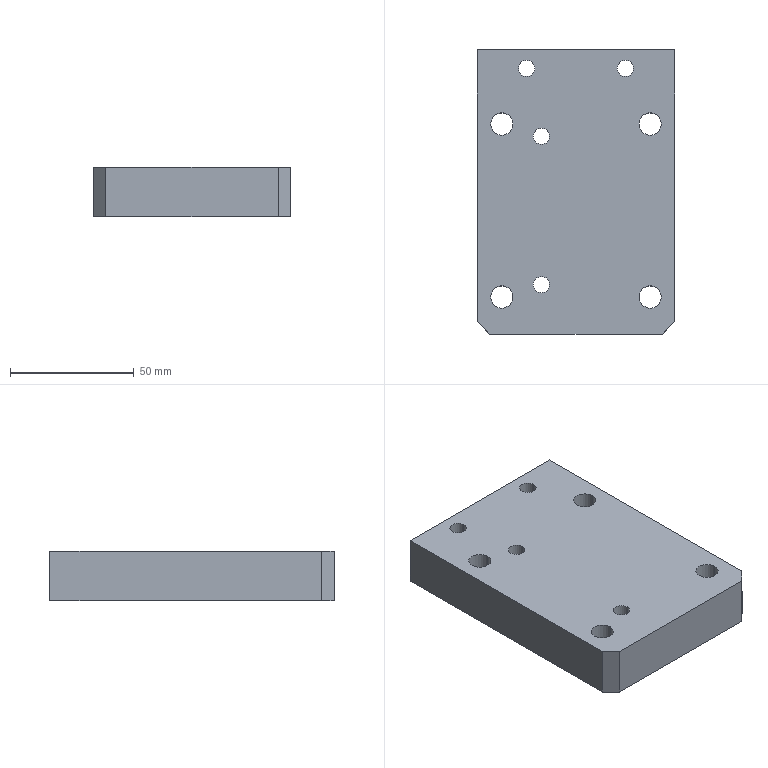Component | SolidWorks | 8TC-A15004-80-02A-2 | 1 solid | 36 faces | box 80 x 115 x 20 mm | volume 174117 mm3 | cylinder 24 | plane 12 | commonest cylinder face diameters 9 x8 11 x8 6.6 x8 | material A3
STEP:
#1=COLOUR_RGB('',0.7922,0.8196,0.9333);
#2=FILL_AREA_STYLE_COLOUR('',#1);
#3=FILL_AREA_STYLE('',(#2));
#4=SURFACE_STYLE_FILL_AREA(#3);
#5=SURFACE_SIDE_STYLE('',(#4));
#6=SURFACE_STYLE_USAGE(.BOTH.,#5);
#7=PRESENTATION_STYLE_ASSIGNMENT((#6));
#8=CARTESIAN_POINT('',(0.2165,-3.642,0.7874));
#9=VERTEX_POINT('',#8);
#10=CARTESIAN_POINT('',(0.5709,-3.642,0.7874));
#11=VERTEX_POINT('',#10);
#12=CARTESIAN_POINT('',(0.3937,-3.642,0.7874));
#13=DIRECTION('',(0.,0.,1.));
#14=DIRECTION('',(1.,0.,0.));
#15=AXIS2_PLACEMENT_3D('',#12,#13,#14);
#16=CIRCLE('',#15,0.1772);
#17=EDGE_CURVE('',#9,#11,#16,.T.);
#18=ORIENTED_EDGE('',*,*,#17,.F.);
#19=CARTESIAN_POINT('',(0.2165,-3.642,1.575));
#20=VERTEX_POINT('',#19);
#21=CARTESIAN_POINT('',(0.2165,-3.642,1.575));
#22=DIRECTION('',(0.,0.,1.));
#23=VECTOR('',#22,39.37);
#24=LINE('',#21,#23);
#25=EDGE_CURVE('',#9,#20,#24,.T.);
#26=ORIENTED_EDGE('',*,*,#25,.T.);
#27=CARTESIAN_POINT('',(0.5709,-3.642,1.575));
#28=VERTEX_POINT('',#27);
#29=CARTESIAN_POINT('',(0.3937,-3.642,1.575));
#30=DIRECTION('',(0.,0.,1.));
#31=DIRECTION('',(1.,0.,0.));
#32=AXIS2_PLACEMENT_3D('',#29,#30,#31);
#33=CIRCLE('',#32,0.1772);
#34=EDGE_CURVE('',#20,#28,#33,.T.);
#35=ORIENTED_EDGE('',*,*,#34,.T.);
#36=CARTESIAN_POINT('',(0.5709,-3.642,1.575));
#37=DIRECTION('',(0.,0.,1.));
#38=VECTOR('',#37,39.37);
#39=LINE('',#36,#38);
#40=EDGE_CURVE('',#11,#28,#39,.T.);
#41=ORIENTED_EDGE('',*,*,#40,.F.);
#42=EDGE_LOOP('',(#18,#26,#35,#41));
#43=FACE_OUTER_BOUND('',#42,.T.);
#44=CARTESIAN_POINT('',(0.3937,-3.642,1.575));
#45=DIRECTION('',(0.,0.,1.));
#46=DIRECTION('',(1.,0.,0.));
#47=AXIS2_PLACEMENT_3D('',#44,#45,#46);
#48=CYLINDRICAL_SURFACE('',#47,0.1772);
#49=ADVANCED_FACE('',(#43),#48,.F.);
#50=CARTESIAN_POINT('',(0.2165,-0.8858,0.7874));
#51=VERTEX_POINT('',#50);
#52=CARTESIAN_POINT('',(0.5709,-0.8858,0.7874));
#53=VERTEX_POINT('',#52);
#54=CARTESIAN_POINT('',(0.3937,-0.8858,0.7874));
#55=DIRECTION('',(0.,0.,1.));
#56=DIRECTION('',(1.,0.,0.));
#57=AXIS2_PLACEMENT_3D('',#54,#55,#56);
#58=CIRCLE('',#57,0.1772);
#59=EDGE_CURVE('',#51,#53,#58,.T.);
#60=ORIENTED_EDGE('',*,*,#59,.F.);
#61=CARTESIAN_POINT('',(0.2165,-0.8858,1.575));
#62=VERTEX_POINT('',#61);
#63=CARTESIAN_POINT('',(0.2165,-0.8858,1.575));
#64=DIRECTION('',(0.,0.,1.));
#65=VECTOR('',#64,39.37);
#66=LINE('',#63,#65);
#67=EDGE_CURVE('',#51,#62,#66,.T.);
#68=ORIENTED_EDGE('',*,*,#67,.T.);
#69=CARTESIAN_POINT('',(0.5709,-0.8858,1.575));
#70=VERTEX_POINT('',#69);
#71=CARTESIAN_POINT('',(0.3937,-0.8858,1.575));
#72=DIRECTION('',(0.,0.,1.));
#73=DIRECTION('',(1.,0.,0.));
#74=AXIS2_PLACEMENT_3D('',#71,#72,#73);
#75=CIRCLE('',#74,0.1772);
#76=EDGE_CURVE('',#62,#70,#75,.T.);
#77=ORIENTED_EDGE('',*,*,#76,.T.);
#78=CARTESIAN_POINT('',(0.5709,-0.8858,1.575));
#79=DIRECTION('',(0.,0.,1.));
#80=VECTOR('',#79,39.37);
#81=LINE('',#78,#80);
#82=EDGE_CURVE('',#53,#70,#81,.T.);
#83=ORIENTED_EDGE('',*,*,#82,.F.);
#84=EDGE_LOOP('',(#60,#68,#77,#83));
#85=FACE_OUTER_BOUND('',#84,.T.);
#86=CARTESIAN_POINT('',(0.3937,-0.8858,1.575));
#87=DIRECTION('',(0.,0.,1.));
#88=DIRECTION('',(1.,0.,0.));
#89=AXIS2_PLACEMENT_3D('',#86,#87,#88);
#90=CYLINDRICAL_SURFACE('',#89,0.1772);
#91=ADVANCED_FACE('',(#85),#90,.F.);
#92=CARTESIAN_POINT('',(2.579,-0.8858,0.7874));
#93=VERTEX_POINT('',#92);
#94=CARTESIAN_POINT('',(2.933,-0.8858,0.7874));
#95=VERTEX_POINT('',#94);
#96=CARTESIAN_POINT('',(2.756,-0.8858,0.7874));
#97=DIRECTION('',(0.,0.,1.));
#98=DIRECTION('',(1.,0.,0.));
#99=AXIS2_PLACEMENT_3D('',#96,#97,#98);
#100=CIRCLE('',#99,0.1772);
#101=EDGE_CURVE('',#93,#95,#100,.T.);
#102=ORIENTED_EDGE('',*,*,#101,.F.);
#103=CARTESIAN_POINT('',(2.579,-0.8858,1.575));
#104=VERTEX_POINT('',#103);
#105=CARTESIAN_POINT('',(2.579,-0.8858,1.575));
#106=DIRECTION('',(0.,0.,1.));
#107=VECTOR('',#106,39.37);
#108=LINE('',#105,#107);
#109=EDGE_CURVE('',#93,#104,#108,.T.);
#110=ORIENTED_EDGE('',*,*,#109,.T.);
#111=CARTESIAN_POINT('',(2.933,-0.8858,1.575));
#112=VERTEX_POINT('',#111);
#113=CARTESIAN_POINT('',(2.756,-0.8858,1.575));
#114=DIRECTION('',(0.,0.,1.));
#115=DIRECTION('',(1.,0.,0.));
#116=AXIS2_PLACEMENT_3D('',#113,#114,#115);
#117=CIRCLE('',#116,0.1772);
#118=EDGE_CURVE('',#104,#112,#117,.T.);
#119=ORIENTED_EDGE('',*,*,#118,.T.);
#120=CARTESIAN_POINT('',(2.933,-0.8858,1.575));
#121=DIRECTION('',(0.,0.,1.));
#122=VECTOR('',#121,39.37);
#123=LINE('',#120,#122);
#124=EDGE_CURVE('',#95,#112,#123,.T.);
#125=ORIENTED_EDGE('',*,*,#124,.F.);
#126=EDGE_LOOP('',(#102,#110,#119,#125));
#127=FACE_OUTER_BOUND('',#126,.T.);
#128=CARTESIAN_POINT('',(2.756,-0.8858,1.575));
#129=DIRECTION('',(0.,0.,1.));
#130=DIRECTION('',(1.,0.,0.));
#131=AXIS2_PLACEMENT_3D('',#128,#129,#130);
#132=CYLINDRICAL_SURFACE('',#131,0.1772);
#133=ADVANCED_FACE('',(#127),#132,.F.);
#134=CARTESIAN_POINT('',(2.579,-3.642,0.7874));
#135=VERTEX_POINT('',#134);
#136=CARTESIAN_POINT('',(2.933,-3.642,0.7874));
#137=VERTEX_POINT('',#136);
#138=CARTESIAN_POINT('',(2.756,-3.642,0.7874));
#139=DIRECTION('',(0.,0.,1.));
#140=DIRECTION('',(1.,0.,0.));
#141=AXIS2_PLACEMENT_3D('',#138,#139,#140);
#142=CIRCLE('',#141,0.1772);
#143=EDGE_CURVE('',#135,#137,#142,.T.);
#144=ORIENTED_EDGE('',*,*,#143,.F.);
#145=CARTESIAN_POINT('',(2.579,-3.642,1.575));
#146=VERTEX_POINT('',#145);
#147=CARTESIAN_POINT('',(2.579,-3.642,1.575));
#148=DIRECTION('',(0.,0.,1.));
#149=VECTOR('',#148,39.37);
#150=LINE('',#147,#149);
#151=EDGE_CURVE('',#135,#146,#150,.T.);
#152=ORIENTED_EDGE('',*,*,#151,.T.);
#153=CARTESIAN_POINT('',(2.933,-3.642,1.575));
#154=VERTEX_POINT('',#153);
#155=CARTESIAN_POINT('',(2.756,-3.642,1.575));
#156=DIRECTION('',(0.,0.,1.));
#157=DIRECTION('',(1.,0.,0.));
#158=AXIS2_PLACEMENT_3D('',#155,#156,#157);
#159=CIRCLE('',#158,0.1772);
#160=EDGE_CURVE('',#146,#154,#159,.T.);
#161=ORIENTED_EDGE('',*,*,#160,.T.);
#162=CARTESIAN_POINT('',(2.933,-3.642,1.575));
#163=DIRECTION('',(0.,0.,1.));
#164=VECTOR('',#163,39.37);
#165=LINE('',#162,#164);
#166=EDGE_CURVE('',#137,#154,#165,.T.);
#167=ORIENTED_EDGE('',*,*,#166,.F.);
#168=EDGE_LOOP('',(#144,#152,#161,#167));
#169=FACE_OUTER_BOUND('',#168,.T.);
#170=CARTESIAN_POINT('',(2.756,-3.642,1.575));
#171=DIRECTION('',(0.,0.,1.));
#172=DIRECTION('',(1.,0.,0.));
#173=AXIS2_PLACEMENT_3D('',#170,#171,#172);
#174=CYLINDRICAL_SURFACE('',#173,0.1772);
#175=ADVANCED_FACE('',(#169),#174,.F.);
#176=CARTESIAN_POINT('',(2.579,0.,1.039));
#177=VERTEX_POINT('',#176);
#178=CARTESIAN_POINT('',(2.146,0.,1.039));
#179=VERTEX_POINT('',#178);
#180=CARTESIAN_POINT('',(2.362,0.,1.039));
#181=DIRECTION('',(0.,0.,-1.));
#182=DIRECTION('',(-1.,0.,0.));
#183=AXIS2_PLACEMENT_3D('',#180,#181,#182);
#184=CIRCLE('',#183,0.2165);
#185=EDGE_CURVE('',#177,#179,#184,.T.);
#186=ORIENTED_EDGE('',*,*,#185,.F.);
#187=CARTESIAN_POINT('',(2.579,0.,0.7874));
#188=VERTEX_POINT('',#187);
#189=CARTESIAN_POINT('',(2.579,0.,0.7874));
#190=DIRECTION('',(0.,0.,-1.));
#191=VECTOR('',#190,39.37);
#192=LINE('',#189,#191);
#193=EDGE_CURVE('',#177,#188,#192,.T.);
#194=ORIENTED_EDGE('',*,*,#193,.T.);
#195=CARTESIAN_POINT('',(2.146,0.,0.7874));
#196=VERTEX_POINT('',#195);
#197=CARTESIAN_POINT('',(2.362,0.,0.7874));
#198=DIRECTION('',(0.,0.,-1.));
#199=DIRECTION('',(-1.,0.,0.));
#200=AXIS2_PLACEMENT_3D('',#197,#198,#199);
#201=CIRCLE('',#200,0.2165);
#202=EDGE_CURVE('',#188,#196,#201,.T.);
#203=ORIENTED_EDGE('',*,*,#202,.T.);
#204=CARTESIAN_POINT('',(2.146,0.,0.7874));
#205=DIRECTION('',(0.,0.,-1.));
#206=VECTOR('',#205,39.37);
#207=LINE('',#204,#206);
#208=EDGE_CURVE('',#179,#196,#207,.T.);
#209=ORIENTED_EDGE('',*,*,#208,.F.);
#210=EDGE_LOOP('',(#186,#194,#203,#209));
#211=FACE_OUTER_BOUND('',#210,.T.);
#212=CARTESIAN_POINT('',(2.362,0.,0.7874));
#213=DIRECTION('',(0.,0.,-1.));
#214=DIRECTION('',(-1.,0.,0.));
#215=AXIS2_PLACEMENT_3D('',#212,#213,#214);
#216=CYLINDRICAL_SURFACE('',#215,0.2165);
#217=ADVANCED_FACE('',(#211),#216,.F.);
#218=CARTESIAN_POINT('',(2.492,0.,1.575));
#219=VERTEX_POINT('',#218);
#220=CARTESIAN_POINT('',(2.232,0.,1.575));
#221=VERTEX_POINT('',#220);
#222=CARTESIAN_POINT('',(2.362,0.,1.575));
#223=DIRECTION('',(0.,0.,-1.));
#224=DIRECTION('',(-1.,0.,0.));
#225=AXIS2_PLACEMENT_3D('',#222,#223,#224);
#226=CIRCLE('',#225,0.1299);
#227=EDGE_CURVE('',#219,#221,#226,.T.);
#228=ORIENTED_EDGE('',*,*,#227,.F.);
#229=CARTESIAN_POINT('',(2.492,0.,1.039));
#230=VERTEX_POINT('',#229);
#231=CARTESIAN_POINT('',(2.492,0.,0.7874));
#232=DIRECTION('',(0.,0.,-1.));
#233=VECTOR('',#232,39.37);
#234=LINE('',#231,#233);
#235=EDGE_CURVE('',#219,#230,#234,.T.);
#236=ORIENTED_EDGE('',*,*,#235,.T.);
#237=CARTESIAN_POINT('',(2.232,0.,1.039));
#238=VERTEX_POINT('',#237);
#239=CARTESIAN_POINT('',(2.362,0.,1.039));
#240=DIRECTION('',(0.,0.,-1.));
#241=DIRECTION('',(-1.,0.,0.));
#242=AXIS2_PLACEMENT_3D('',#239,#240,#241);
#243=CIRCLE('',#242,0.1299);
#244=EDGE_CURVE('',#230,#238,#243,.T.);
#245=ORIENTED_EDGE('',*,*,#244,.T.);
#246=CARTESIAN_POINT('',(2.232,0.,0.7874));
#247=DIRECTION('',(0.,0.,-1.));
#248=VECTOR('',#247,39.37);
#249=LINE('',#246,#248);
#250=EDGE_CURVE('',#221,#238,#249,.T.);
#251=ORIENTED_EDGE('',*,*,#250,.F.);
#252=EDGE_LOOP('',(#228,#236,#245,#251));
#253=FACE_OUTER_BOUND('',#252,.T.);
#254=CARTESIAN_POINT('',(2.362,0.,0.7874));
#255=DIRECTION('',(0.,0.,-1.));
#256=DIRECTION('',(-1.,0.,0.));
#257=AXIS2_PLACEMENT_3D('',#254,#255,#256);
#258=CYLINDRICAL_SURFACE('',#257,0.1299);
#259=ADVANCED_FACE('',(#253),#258,.F.);
#260=CARTESIAN_POINT('',(1.004,0.,1.039));
#261=VERTEX_POINT('',#260);
#262=CARTESIAN_POINT('',(0.5709,0.,1.039));
#263=VERTEX_POINT('',#262);
#264=CARTESIAN_POINT('',(0.7874,0.,1.039));
#265=DIRECTION('',(0.,0.,-1.));
#266=DIRECTION('',(-1.,0.,0.));
#267=AXIS2_PLACEMENT_3D('',#264,#265,#266);
#268=CIRCLE('',#267,0.2165);
#269=EDGE_CURVE('',#261,#263,#268,.T.);
#270=ORIENTED_EDGE('',*,*,#269,.F.);
#271=CARTESIAN_POINT('',(1.004,0.,0.7874));
#272=VERTEX_POINT('',#271);
#273=CARTESIAN_POINT('',(1.004,0.,0.7874));
#274=DIRECTION('',(0.,0.,-1.));
#275=VECTOR('',#274,39.37);
#276=LINE('',#273,#275);
#277=EDGE_CURVE('',#261,#272,#276,.T.);
#278=ORIENTED_EDGE('',*,*,#277,.T.);
#279=CARTESIAN_POINT('',(0.5709,0.,0.7874));
#280=VERTEX_POINT('',#279);
#281=CARTESIAN_POINT('',(0.7874,0.,0.7874));
#282=DIRECTION('',(0.,0.,-1.));
#283=DIRECTION('',(-1.,0.,0.));
#284=AXIS2_PLACEMENT_3D('',#281,#282,#283);
#285=CIRCLE('',#284,0.2165);
#286=EDGE_CURVE('',#272,#280,#285,.T.);
#287=ORIENTED_EDGE('',*,*,#286,.T.);
#288=CARTESIAN_POINT('',(0.5709,0.,0.7874));
#289=DIRECTION('',(0.,0.,-1.));
#290=VECTOR('',#289,39.37);
#291=LINE('',#288,#290);
#292=EDGE_CURVE('',#263,#280,#291,.T.);
#293=ORIENTED_EDGE('',*,*,#292,.F.);
#294=EDGE_LOOP('',(#270,#278,#287,#293));
#295=FACE_OUTER_BOUND('',#294,.T.);
#296=CARTESIAN_POINT('',(0.7874,0.,0.7874));
#297=DIRECTION('',(0.,0.,-1.));
#298=DIRECTION('',(-1.,0.,0.));
#299=AXIS2_PLACEMENT_3D('',#296,#297,#298);
#300=CYLINDRICAL_SURFACE('',#299,0.2165);
#301=ADVANCED_FACE('',(#295),#300,.F.);
#302=CARTESIAN_POINT('',(0.9173,0.,1.575));
#303=VERTEX_POINT('',#302);
#304=CARTESIAN_POINT('',(0.6575,0.,1.575));
#305=VERTEX_POINT('',#304);
#306=CARTESIAN_POINT('',(0.7874,0.,1.575));
#307=DIRECTION('',(0.,0.,-1.));
#308=DIRECTION('',(-1.,0.,0.));
#309=AXIS2_PLACEMENT_3D('',#306,#307,#308);
#310=CIRCLE('',#309,0.1299);
#311=EDGE_CURVE('',#303,#305,#310,.T.);
#312=ORIENTED_EDGE('',*,*,#311,.F.);
#313=CARTESIAN_POINT('',(0.9173,0.,1.039));
#314=VERTEX_POINT('',#313);
#315=CARTESIAN_POINT('',(0.9173,0.,0.7874));
#316=DIRECTION('',(0.,0.,-1.));
#317=VECTOR('',#316,39.37);
#318=LINE('',#315,#317);
#319=EDGE_CURVE('',#303,#314,#318,.T.);
#320=ORIENTED_EDGE('',*,*,#319,.T.);
#321=CARTESIAN_POINT('',(0.6575,0.,1.039));
#322=VERTEX_POINT('',#321);
#323=CARTESIAN_POINT('',(0.7874,0.,1.039));
#324=DIRECTION('',(0.,0.,-1.));
#325=DIRECTION('',(-1.,0.,0.));
#326=AXIS2_PLACEMENT_3D('',#323,#324,#325);
#327=CIRCLE('',#326,0.1299);
#328=EDGE_CURVE('',#314,#322,#327,.T.);
#329=ORIENTED_EDGE('',*,*,#328,.T.);
#330=CARTESIAN_POINT('',(0.6575,0.,0.7874));
#331=DIRECTION('',(0.,0.,-1.));
#332=VECTOR('',#331,39.37);
#333=LINE('',#330,#332);
#334=EDGE_CURVE('',#305,#322,#333,.T.);
#335=ORIENTED_EDGE('',*,*,#334,.F.);
#336=EDGE_LOOP('',(#312,#320,#329,#335));
#337=FACE_OUTER_BOUND('',#336,.T.);
#338=CARTESIAN_POINT('',(0.7874,0.,0.7874));
#339=DIRECTION('',(0.,0.,-1.));
#340=DIRECTION('',(-1.,0.,0.));
#341=AXIS2_PLACEMENT_3D('',#338,#339,#340);
#342=CYLINDRICAL_SURFACE('',#341,0.1299);
#343=ADVANCED_FACE('',(#337),#342,.F.);
#344=CARTESIAN_POINT('',(1.24,-1.083,1.039));
#345=VERTEX_POINT('',#344);
#346=CARTESIAN_POINT('',(0.8071,-1.083,1.039));
#347=VERTEX_POINT('',#346);
#348=CARTESIAN_POINT('',(1.024,-1.083,1.039));
#349=DIRECTION('',(0.,0.,-1.));
#350=DIRECTION('',(-1.,0.,0.));
#351=AXIS2_PLACEMENT_3D('',#348,#349,#350);
#352=CIRCLE('',#351,0.2165);
#353=EDGE_CURVE('',#345,#347,#352,.T.);
#354=ORIENTED_EDGE('',*,*,#353,.F.);
#355=CARTESIAN_POINT('',(1.24,-1.083,0.7874));
#356=VERTEX_POINT('',#355);
#357=CARTESIAN_POINT('',(1.24,-1.083,0.7874));
#358=DIRECTION('',(0.,0.,-1.));
#359=VECTOR('',#358,39.37);
#360=LINE('',#357,#359);
#361=EDGE_CURVE('',#345,#356,#360,.T.);
#362=ORIENTED_EDGE('',*,*,#361,.T.);
#363=CARTESIAN_POINT('',(0.8071,-1.083,0.7874));
#364=VERTEX_POINT('',#363);
#365=CARTESIAN_POINT('',(1.024,-1.083,0.7874));
#366=DIRECTION('',(0.,0.,-1.));
#367=DIRECTION('',(-1.,0.,0.));
#368=AXIS2_PLACEMENT_3D('',#365,#366,#367);
#369=CIRCLE('',#368,0.2165);
#370=EDGE_CURVE('',#356,#364,#369,.T.);
#371=ORIENTED_EDGE('',*,*,#370,.T.);
#372=CARTESIAN_POINT('',(0.8071,-1.083,0.7874));
#373=DIRECTION('',(0.,0.,-1.));
#374=VECTOR('',#373,39.37);
#375=LINE('',#372,#374);
#376=EDGE_CURVE('',#347,#364,#375,.T.);
#377=ORIENTED_EDGE('',*,*,#376,.F.);
#378=EDGE_LOOP('',(#354,#362,#371,#377));
#379=FACE_OUTER_BOUND('',#378,.T.);
#380=CARTESIAN_POINT('',(1.024,-1.083,0.7874));
#381=DIRECTION('',(0.,0.,-1.));
#382=DIRECTION('',(-1.,0.,0.));
#383=AXIS2_PLACEMENT_3D('',#380,#381,#382);
#384=CYLINDRICAL_SURFACE('',#383,0.2165);
#385=ADVANCED_FACE('',(#379),#384,.F.);
#386=CARTESIAN_POINT('',(1.154,-1.083,1.575));
#387=VERTEX_POINT('',#386);
#388=CARTESIAN_POINT('',(0.8937,-1.083,1.575));
#389=VERTEX_POINT('',#388);
#390=CARTESIAN_POINT('',(1.024,-1.083,1.575));
#391=DIRECTION('',(0.,0.,-1.));
#392=DIRECTION('',(-1.,0.,0.));
#393=AXIS2_PLACEMENT_3D('',#390,#391,#392);
#394=CIRCLE('',#393,0.1299);
#395=EDGE_CURVE('',#387,#389,#394,.T.);
#396=ORIENTED_EDGE('',*,*,#395,.F.);
#397=CARTESIAN_POINT('',(1.154,-1.083,1.039));
#398=VERTEX_POINT('',#397);
#399=CARTESIAN_POINT('',(1.154,-1.083,0.7874));
#400=DIRECTION('',(0.,0.,-1.));
#401=VECTOR('',#400,39.37);
#402=LINE('',#399,#401);
#403=EDGE_CURVE('',#387,#398,#402,.T.);
#404=ORIENTED_EDGE('',*,*,#403,.T.);
#405=CARTESIAN_POINT('',(0.8937,-1.083,1.039));
#406=VERTEX_POINT('',#405);
#407=CARTESIAN_POINT('',(1.024,-1.083,1.039));
#408=DIRECTION('',(0.,0.,-1.));
#409=DIRECTION('',(-1.,0.,0.));
#410=AXIS2_PLACEMENT_3D('',#407,#408,#409);
#411=CIRCLE('',#410,0.1299);
#412=EDGE_CURVE('',#398,#406,#411,.T.);
#413=ORIENTED_EDGE('',*,*,#412,.T.);
#414=CARTESIAN_POINT('',(0.8937,-1.083,0.7874));
#415=DIRECTION('',(0.,0.,-1.));
#416=VECTOR('',#415,39.37);
#417=LINE('',#414,#416);
#418=EDGE_CURVE('',#389,#406,#417,.T.);
#419=ORIENTED_EDGE('',*,*,#418,.F.);
#420=EDGE_LOOP('',(#396,#404,#413,#419));
#421=FACE_OUTER_BOUND('',#420,.T.);
#422=CARTESIAN_POINT('',(1.024,-1.083,0.7874));
#423=DIRECTION('',(0.,0.,-1.));
#424=DIRECTION('',(-1.,0.,0.));
#425=AXIS2_PLACEMENT_3D('',#422,#423,#424);
#426=CYLINDRICAL_SURFACE('',#425,0.1299);
#427=ADVANCED_FACE('',(#421),#426,.F.);
#428=CARTESIAN_POINT('',(1.24,-3.445,1.039));
#429=VERTEX_POINT('',#428);
#430=CARTESIAN_POINT('',(0.8071,-3.445,1.039));
#431=VERTEX_POINT('',#430);
#432=CARTESIAN_POINT('',(1.024,-3.445,1.039));
#433=DIRECTION('',(0.,0.,-1.));
#434=DIRECTION('',(-1.,0.,0.));
#435=AXIS2_PLACEMENT_3D('',#432,#433,#434);
#436=CIRCLE('',#435,0.2165);
#437=EDGE_CURVE('',#429,#431,#436,.T.);
#438=ORIENTED_EDGE('',*,*,#437,.F.);
#439=CARTESIAN_POINT('',(1.24,-3.445,0.7874));
#440=VERTEX_POINT('',#439);
#441=CARTESIAN_POINT('',(1.24,-3.445,0.7874));
#442=DIRECTION('',(0.,0.,-1.));
#443=VECTOR('',#442,39.37);
#444=LINE('',#441,#443);
#445=EDGE_CURVE('',#429,#440,#444,.T.);
#446=ORIENTED_EDGE('',*,*,#445,.T.);
#447=CARTESIAN_POINT('',(0.8071,-3.445,0.7874));
#448=VERTEX_POINT('',#447);
#449=CARTESIAN_POINT('',(1.024,-3.445,0.7874));
#450=DIRECTION('',(0.,0.,-1.));
#451=DIRECTION('',(-1.,0.,0.));
#452=AXIS2_PLACEMENT_3D('',#449,#450,#451);
#453=CIRCLE('',#452,0.2165);
#454=EDGE_CURVE('',#440,#448,#453,.T.);
#455=ORIENTED_EDGE('',*,*,#454,.T.);
#456=CARTESIAN_POINT('',(0.8071,-3.445,0.7874));
#457=DIRECTION('',(0.,0.,-1.));
#458=VECTOR('',#457,39.37);
#459=LINE('',#456,#458);
#460=EDGE_CURVE('',#431,#448,#459,.T.);
#461=ORIENTED_EDGE('',*,*,#460,.F.);
#462=EDGE_LOOP('',(#438,#446,#455,#461));
#463=FACE_OUTER_BOUND('',#462,.T.);
#464=CARTESIAN_POINT('',(1.024,-3.445,0.7874));
#465=DIRECTION('',(0.,0.,-1.));
#466=DIRECTION('',(-1.,0.,0.));
#467=AXIS2_PLACEMENT_3D('',#464,#465,#466);
#468=CYLINDRICAL_SURFACE('',#467,0.2165);
#469=ADVANCED_FACE('',(#463),#468,.F.);
#470=CARTESIAN_POINT('',(1.154,-3.445,1.575));
#471=VERTEX_POINT('',#470);
#472=CARTESIAN_POINT('',(0.8937,-3.445,1.575));
#473=VERTEX_POINT('',#472);
#474=CARTESIAN_POINT('',(1.024,-3.445,1.575));
#475=DIRECTION('',(0.,0.,-1.));
#476=DIRECTION('',(-1.,0.,0.));
#477=AXIS2_PLACEMENT_3D('',#474,#475,#476);
#478=CIRCLE('',#477,0.1299);
#479=EDGE_CURVE('',#471,#473,#478,.T.);
#480=ORIENTED_EDGE('',*,*,#479,.F.);
#481=CARTESIAN_POINT('',(1.154,-3.445,1.039));
#482=VERTEX_POINT('',#481);
#483=CARTESIAN_POINT('',(1.154,-3.445,0.7874));
#484=DIRECTION('',(0.,0.,-1.));
#485=VECTOR('',#484,39.37);
#486=LINE('',#483,#485);
#487=EDGE_CURVE('',#471,#482,#486,.T.);
#488=ORIENTED_EDGE('',*,*,#487,.T.);
#489=CARTESIAN_POINT('',(0.8937,-3.445,1.039));
#490=VERTEX_POINT('',#489);
#491=CARTESIAN_POINT('',(1.024,-3.445,1.039));
#492=DIRECTION('',(0.,0.,-1.));
#493=DIRECTION('',(-1.,0.,0.));
#494=AXIS2_PLACEMENT_3D('',#491,#492,#493);
#495=CIRCLE('',#494,0.1299);
#496=EDGE_CURVE('',#482,#490,#495,.T.);
#497=ORIENTED_EDGE('',*,*,#496,.T.);
#498=CARTESIAN_POINT('',(0.8937,-3.445,0.7874));
#499=DIRECTION('',(0.,0.,-1.));
#500=VECTOR('',#499,39.37);
#501=LINE('',#498,#500);
#502=EDGE_CURVE('',#473,#490,#501,.T.);
#503=ORIENTED_EDGE('',*,*,#502,.F.);
#504=EDGE_LOOP('',(#480,#488,#497,#503));
#505=FACE_OUTER_BOUND('',#504,.T.);
#506=CARTESIAN_POINT('',(1.024,-3.445,0.7874));
#507=DIRECTION('',(0.,0.,-1.));
#508=DIRECTION('',(-1.,0.,0.));
#509=AXIS2_PLACEMENT_3D('',#506,#507,#508);
#510=CYLINDRICAL_SURFACE('',#509,0.1299);
#511=ADVANCED_FACE('',(#505),#510,.F.);
#512=CARTESIAN_POINT('',(0.3937,-3.642,1.575));
#513=DIRECTION('',(0.,0.,1.));
#514=DIRECTION('',(1.,0.,0.));
#515=AXIS2_PLACEMENT_3D('',#512,#513,#514);
#516=CIRCLE('',#515,0.1772);
#517=EDGE_CURVE('',#28,#20,#516,.T.);
#518=ORIENTED_EDGE('',*,*,#517,.F.);
#519=ORIENTED_EDGE('',*,*,#34,.F.);
#520=EDGE_LOOP('',(#518,#519));
#521=FACE_BOUND('',#520,.T.);
#522=CARTESIAN_POINT('',(0.3937,-0.8858,1.575));
#523=DIRECTION('',(0.,0.,1.));
#524=DIRECTION('',(1.,0.,0.));
#525=AXIS2_PLACEMENT_3D('',#522,#523,#524);
#526=CIRCLE('',#525,0.1772);
#527=EDGE_CURVE('',#70,#62,#526,.T.);
#528=ORIENTED_EDGE('',*,*,#527,.F.);
#529=ORIENTED_EDGE('',*,*,#76,.F.);
#530=EDGE_LOOP('',(#528,#529));
#531=FACE_BOUND('',#530,.T.);
#532=CARTESIAN_POINT('',(2.756,-0.8858,1.575));
#533=DIRECTION('',(0.,0.,1.));
#534=DIRECTION('',(1.,0.,0.));
#535=AXIS2_PLACEMENT_3D('',#532,#533,#534);
#536=CIRCLE('',#535,0.1772);
#537=EDGE_CURVE('',#112,#104,#536,.T.);
#538=ORIENTED_EDGE('',*,*,#537,.F.);
#539=ORIENTED_EDGE('',*,*,#118,.F.);
#540=EDGE_LOOP('',(#538,#539));
#541=FACE_BOUND('',#540,.T.);
#542=CARTESIAN_POINT('',(2.362,0.,1.575));
#543=DIRECTION('',(0.,0.,-1.));
#544=DIRECTION('',(-1.,0.,0.));
#545=AXIS2_PLACEMENT_3D('',#542,#543,#544);
#546=CIRCLE('',#545,0.1299);
#547=EDGE_CURVE('',#221,#219,#546,.T.);
#548=ORIENTED_EDGE('',*,*,#547,.T.);
#549=ORIENTED_EDGE('',*,*,#227,.T.);
#550=EDGE_LOOP('',(#548,#549));
#551=FACE_BOUND('',#550,.T.);
#552=CARTESIAN_POINT('',(0.7874,0.,1.575));
#553=DIRECTION('',(0.,0.,-1.));
#554=DIRECTION('',(-1.,0.,0.));
#555=AXIS2_PLACEMENT_3D('',#552,#553,#554);
#556=CIRCLE('',#555,0.1299);
#557=EDGE_CURVE('',#305,#303,#556,.T.);
#558=ORIENTED_EDGE('',*,*,#557,.T.);
#559=ORIENTED_EDGE('',*,*,#311,.T.);
#560=EDGE_LOOP('',(#558,#559));
#561=FACE_BOUND('',#560,.T.);
#562=CARTESIAN_POINT('',(1.024,-1.083,1.575));
#563=DIRECTION('',(0.,0.,-1.));
#564=DIRECTION('',(-1.,0.,0.));
#565=AXIS2_PLACEMENT_3D('',#562,#563,#564);
#566=CIRCLE('',#565,0.1299);
#567=EDGE_CURVE('',#389,#387,#566,.T.);
#568=ORIENTED_EDGE('',*,*,#567,.T.);
#569=ORIENTED_EDGE('',*,*,#395,.T.);
#570=EDGE_LOOP('',(#568,#569));
#571=FACE_BOUND('',#570,.T.);
#572=CARTESIAN_POINT('',(1.024,-3.445,1.575));
#573=DIRECTION('',(0.,0.,-1.));
#574=DIRECTION('',(-1.,0.,0.));
#575=AXIS2_PLACEMENT_3D('',#572,#573,#574);
#576=CIRCLE('',#575,0.1299);
#577=EDGE_CURVE('',#473,#471,#576,.T.);
#578=ORIENTED_EDGE('',*,*,#577,.T.);
#579=ORIENTED_EDGE('',*,*,#479,.T.);
#580=EDGE_LOOP('',(#578,#579));
#581=FACE_BOUND('',#580,.T.);
#582=CARTESIAN_POINT('',(0.1969,-4.232,1.575));
#583=VERTEX_POINT('',#582);
#584=CARTESIAN_POINT('',(2.953,-4.232,1.575));
#585=VERTEX_POINT('',#584);
#586=CARTESIAN_POINT('',(3.15,-4.232,1.575));
#587=DIRECTION('',(1.,0.,0.));
#588=VECTOR('',#587,39.37);
#589=LINE('',#586,#588);
#590=EDGE_CURVE('',#583,#585,#589,.T.);
#591=ORIENTED_EDGE('',*,*,#590,.T.);
#592=CARTESIAN_POINT('',(3.15,-4.035,1.575));
#593=VERTEX_POINT('',#592);
#594=CARTESIAN_POINT('',(3.15,-4.035,1.575));
#595=DIRECTION('',(0.7071,0.7071,0.));
#596=VECTOR('',#595,39.37);
#597=LINE('',#594,#596);
#598=EDGE_CURVE('',#585,#593,#597,.T.);
#599=ORIENTED_EDGE('',*,*,#598,.T.);
#600=CARTESIAN_POINT('',(3.15,0.2953,1.575));
#601=VERTEX_POINT('',#600);
#602=CARTESIAN_POINT('',(3.15,-4.232,1.575));
#603=DIRECTION('',(-0.,1.,0.));
#604=VECTOR('',#603,39.37);
#605=LINE('',#602,#604);
#606=EDGE_CURVE('',#593,#601,#605,.T.);
#607=ORIENTED_EDGE('',*,*,#606,.T.);
#608=CARTESIAN_POINT('',(0.,0.2953,1.575));
#609=VERTEX_POINT('',#608);
#610=CARTESIAN_POINT('',(3.15,0.2953,1.575));
#611=DIRECTION('',(-1.,0.,0.));
#612=VECTOR('',#611,39.37);
#613=LINE('',#610,#612);
#614=EDGE_CURVE('',#601,#609,#613,.T.);
#615=ORIENTED_EDGE('',*,*,#614,.T.);
#616=CARTESIAN_POINT('',(0.,-4.035,1.575));
#617=VERTEX_POINT('',#616);
#618=CARTESIAN_POINT('',(0.,-4.232,1.575));
#619=DIRECTION('',(0.,-1.,0.));
#620=VECTOR('',#619,39.37);
#621=LINE('',#618,#620);
#622=EDGE_CURVE('',#609,#617,#621,.T.);
#623=ORIENTED_EDGE('',*,*,#622,.T.);
#624=CARTESIAN_POINT('',(0.1969,-4.232,1.575));
#625=DIRECTION('',(0.7071,-0.7071,0.));
#626=VECTOR('',#625,39.37);
#627=LINE('',#624,#626);
#628=EDGE_CURVE('',#617,#583,#627,.T.);
#629=ORIENTED_EDGE('',*,*,#628,.T.);
#630=EDGE_LOOP('',(#591,#599,#607,#615,#623,#629));
#631=FACE_OUTER_BOUND('',#630,.T.);
#632=CARTESIAN_POINT('',(2.756,-3.642,1.575));
#633=DIRECTION('',(0.,0.,1.));
#634=DIRECTION('',(1.,0.,0.));
#635=AXIS2_PLACEMENT_3D('',#632,#633,#634);
#636=CIRCLE('',#635,0.1772);
#637=EDGE_CURVE('',#154,#146,#636,.T.);
#638=ORIENTED_EDGE('',*,*,#637,.F.);
#639=ORIENTED_EDGE('',*,*,#160,.F.);
#640=EDGE_LOOP('',(#638,#639));
#641=FACE_BOUND('',#640,.T.);
#642=CARTESIAN_POINT('',(1.575,-1.969,1.575));
#643=DIRECTION('',(0.,0.,-1.));
#644=DIRECTION('',(-1.,0.,0.));
#645=AXIS2_PLACEMENT_3D('',#642,#643,#644);
#646=PLANE('',#645);
#647=ADVANCED_FACE('',(#521,#531,#541,#551,#561,#571,#581,#631,#641),#646,.F.);
#648=CARTESIAN_POINT('',(3.15,0.2953,0.7874));
#649=VERTEX_POINT('',#648);
#650=CARTESIAN_POINT('',(0.,0.2953,0.7874));
#651=VERTEX_POINT('',#650);
#652=CARTESIAN_POINT('',(3.15,0.2953,0.7874));
#653=DIRECTION('',(-1.,0.,0.));
#654=VECTOR('',#653,39.37);
#655=LINE('',#652,#654);
#656=EDGE_CURVE('',#649,#651,#655,.T.);
#657=ORIENTED_EDGE('',*,*,#656,.T.);
#658=CARTESIAN_POINT('',(0.,0.2953,1.575));
#659=DIRECTION('',(0.,0.,-1.));
#660=VECTOR('',#659,39.37);
#661=LINE('',#658,#660);
#662=EDGE_CURVE('',#609,#651,#661,.T.);
#663=ORIENTED_EDGE('',*,*,#662,.F.);
#664=ORIENTED_EDGE('',*,*,#614,.F.);
#665=CARTESIAN_POINT('',(3.15,0.2953,1.575));
#666=DIRECTION('',(0.,0.,-1.));
#667=VECTOR('',#666,39.37);
#668=LINE('',#665,#667);
#669=EDGE_CURVE('',#601,#649,#668,.T.);
#670=ORIENTED_EDGE('',*,*,#669,.T.);
#671=EDGE_LOOP('',(#657,#663,#664,#670));
#672=FACE_OUTER_BOUND('',#671,.T.);
#673=CARTESIAN_POINT('',(3.15,0.2953,1.575));
#674=DIRECTION('',(0.,-1.,0.));
#675=DIRECTION('',(1.,0.,0.));
#676=AXIS2_PLACEMENT_3D('',#673,#674,#675);
#677=PLANE('',#676);
#678=ADVANCED_FACE('',(#672),#677,.F.);
#679=CARTESIAN_POINT('',(0.,-4.035,0.7874));
#680=VERTEX_POINT('',#679);
#681=CARTESIAN_POINT('',(0.,-4.232,0.7874));
#682=DIRECTION('',(0.,-1.,0.));
#683=VECTOR('',#682,39.37);
#684=LINE('',#681,#683);
#685=EDGE_CURVE('',#651,#680,#684,.T.);
#686=ORIENTED_EDGE('',*,*,#685,.T.);
#687=CARTESIAN_POINT('',(0.,-4.035,1.575));
#688=DIRECTION('',(0.,0.,1.));
#689=VECTOR('',#688,39.37);
#690=LINE('',#687,#689);
#691=EDGE_CURVE('',#680,#617,#690,.T.);
#692=ORIENTED_EDGE('',*,*,#691,.T.);
#693=ORIENTED_EDGE('',*,*,#622,.F.);
#694=ORIENTED_EDGE('',*,*,#662,.T.);
#695=EDGE_LOOP('',(#686,#692,#693,#694));
#696=FACE_OUTER_BOUND('',#695,.T.);
#697=CARTESIAN_POINT('',(0.,-4.232,1.575));
#698=DIRECTION('',(1.,0.,0.));
#699=DIRECTION('',(-0.,1.,0.));
#700=AXIS2_PLACEMENT_3D('',#697,#698,#699);
#701=PLANE('',#700);
#702=ADVANCED_FACE('',(#696),#701,.F.);
#703=CARTESIAN_POINT('',(0.1969,-4.232,0.7874));
#704=VERTEX_POINT('',#703);
#705=CARTESIAN_POINT('',(2.953,-4.232,0.7874));
#706=VERTEX_POINT('',#705);
#707=CARTESIAN_POINT('',(3.15,-4.232,0.7874));
#708=DIRECTION('',(1.,0.,0.));
#709=VECTOR('',#708,39.37);
#710=LINE('',#707,#709);
#711=EDGE_CURVE('',#704,#706,#710,.T.);
#712=ORIENTED_EDGE('',*,*,#711,.T.);
#713=CARTESIAN_POINT('',(2.953,-4.232,1.575));
#714=DIRECTION('',(0.,0.,1.));
#715=VECTOR('',#714,39.37);
#716=LINE('',#713,#715);
#717=EDGE_CURVE('',#706,#585,#716,.T.);
#718=ORIENTED_EDGE('',*,*,#717,.T.);
#719=ORIENTED_EDGE('',*,*,#590,.F.);
#720=CARTESIAN_POINT('',(0.1969,-4.232,1.575));
#721=DIRECTION('',(0.,0.,-1.));
#722=VECTOR('',#721,39.37);
#723=LINE('',#720,#722);
#724=EDGE_CURVE('',#583,#704,#723,.T.);
#725=ORIENTED_EDGE('',*,*,#724,.T.);
#726=EDGE_LOOP('',(#712,#718,#719,#725));
#727=FACE_OUTER_BOUND('',#726,.T.);
#728=CARTESIAN_POINT('',(3.15,-4.232,1.575));
#729=DIRECTION('',(0.,1.,0.));
#730=DIRECTION('',(-1.,0.,0.));
#731=AXIS2_PLACEMENT_3D('',#728,#729,#730);
#732=PLANE('',#731);
#733=ADVANCED_FACE('',(#727),#732,.F.);
#734=ORIENTED_EDGE('',*,*,#606,.F.);
#735=CARTESIAN_POINT('',(3.15,-4.035,0.7874));
#736=VERTEX_POINT('',#735);
#737=CARTESIAN_POINT('',(3.15,-4.035,1.575));
#738=DIRECTION('',(0.,0.,-1.));
#739=VECTOR('',#738,39.37);
#740=LINE('',#737,#739);
#741=EDGE_CURVE('',#593,#736,#740,.T.);
#742=ORIENTED_EDGE('',*,*,#741,.T.);
#743=CARTESIAN_POINT('',(3.15,-4.232,0.7874));
#744=DIRECTION('',(-0.,1.,0.));
#745=VECTOR('',#744,39.37);
#746=LINE('',#743,#745);
#747=EDGE_CURVE('',#736,#649,#746,.T.);
#748=ORIENTED_EDGE('',*,*,#747,.T.);
#749=ORIENTED_EDGE('',*,*,#669,.F.);
#750=EDGE_LOOP('',(#734,#742,#748,#749));
#751=FACE_OUTER_BOUND('',#750,.T.);
#752=CARTESIAN_POINT('',(3.15,-4.232,1.575));
#753=DIRECTION('',(-1.,-0.,0.));
#754=DIRECTION('',(0.,-1.,0.));
#755=AXIS2_PLACEMENT_3D('',#752,#753,#754);
#756=PLANE('',#755);
#757=ADVANCED_FACE('',(#751),#756,.F.);
#758=CARTESIAN_POINT('',(0.3937,-3.642,0.7874));
#759=DIRECTION('',(0.,0.,1.));
#760=DIRECTION('',(1.,0.,0.));
#761=AXIS2_PLACEMENT_3D('',#758,#759,#760);
#762=CIRCLE('',#761,0.1772);
#763=EDGE_CURVE('',#11,#9,#762,.T.);
#764=ORIENTED_EDGE('',*,*,#763,.T.);
#765=ORIENTED_EDGE('',*,*,#17,.T.);
#766=EDGE_LOOP('',(#764,#765));
#767=FACE_BOUND('',#766,.T.);
#768=CARTESIAN_POINT('',(0.3937,-0.8858,0.7874));
#769=DIRECTION('',(0.,0.,1.));
#770=DIRECTION('',(1.,0.,0.));
#771=AXIS2_PLACEMENT_3D('',#768,#769,#770);
#772=CIRCLE('',#771,0.1772);
#773=EDGE_CURVE('',#53,#51,#772,.T.);
#774=ORIENTED_EDGE('',*,*,#773,.T.);
#775=ORIENTED_EDGE('',*,*,#59,.T.);
#776=EDGE_LOOP('',(#774,#775));
#777=FACE_BOUND('',#776,.T.);
#778=CARTESIAN_POINT('',(2.756,-0.8858,0.7874));
#779=DIRECTION('',(0.,0.,1.));
#780=DIRECTION('',(1.,0.,0.));
#781=AXIS2_PLACEMENT_3D('',#778,#779,#780);
#782=CIRCLE('',#781,0.1772);
#783=EDGE_CURVE('',#95,#93,#782,.T.);
#784=ORIENTED_EDGE('',*,*,#783,.T.);
#785=ORIENTED_EDGE('',*,*,#101,.T.);
#786=EDGE_LOOP('',(#784,#785));
#787=FACE_BOUND('',#786,.T.);
#788=CARTESIAN_POINT('',(2.756,-3.642,0.7874));
#789=DIRECTION('',(0.,0.,1.));
#790=DIRECTION('',(1.,0.,0.));
#791=AXIS2_PLACEMENT_3D('',#788,#789,#790);
#792=CIRCLE('',#791,0.1772);
#793=EDGE_CURVE('',#137,#135,#792,.T.);
#794=ORIENTED_EDGE('',*,*,#793,.T.);
#795=ORIENTED_EDGE('',*,*,#143,.T.);
#796=EDGE_LOOP('',(#794,#795));
#797=FACE_BOUND('',#796,.T.);
#798=CARTESIAN_POINT('',(2.362,0.,0.7874));
#799=DIRECTION('',(0.,0.,-1.));
#800=DIRECTION('',(-1.,0.,0.));
#801=AXIS2_PLACEMENT_3D('',#798,#799,#800);
#802=CIRCLE('',#801,0.2165);
#803=EDGE_CURVE('',#196,#188,#802,.T.);
#804=ORIENTED_EDGE('',*,*,#803,.F.);
#805=ORIENTED_EDGE('',*,*,#202,.F.);
#806=EDGE_LOOP('',(#804,#805));
#807=FACE_BOUND('',#806,.T.);
#808=CARTESIAN_POINT('',(0.7874,0.,0.7874));
#809=DIRECTION('',(0.,0.,-1.));
#810=DIRECTION('',(-1.,0.,0.));
#811=AXIS2_PLACEMENT_3D('',#808,#809,#810);
#812=CIRCLE('',#811,0.2165);
#813=EDGE_CURVE('',#280,#272,#812,.T.);
#814=ORIENTED_EDGE('',*,*,#813,.F.);
#815=ORIENTED_EDGE('',*,*,#286,.F.);
#816=EDGE_LOOP('',(#814,#815));
#817=FACE_BOUND('',#816,.T.);
#818=CARTESIAN_POINT('',(1.024,-1.083,0.7874));
#819=DIRECTION('',(0.,0.,-1.));
#820=DIRECTION('',(-1.,0.,0.));
#821=AXIS2_PLACEMENT_3D('',#818,#819,#820);
#822=CIRCLE('',#821,0.2165);
#823=EDGE_CURVE('',#364,#356,#822,.T.);
#824=ORIENTED_EDGE('',*,*,#823,.F.);
#825=ORIENTED_EDGE('',*,*,#370,.F.);
#826=EDGE_LOOP('',(#824,#825));
#827=FACE_BOUND('',#826,.T.);
#828=CARTESIAN_POINT('',(1.024,-3.445,0.7874));
#829=DIRECTION('',(0.,0.,-1.));
#830=DIRECTION('',(-1.,0.,0.));
#831=AXIS2_PLACEMENT_3D('',#828,#829,#830);
#832=CIRCLE('',#831,0.2165);
#833=EDGE_CURVE('',#448,#440,#832,.T.);
#834=ORIENTED_EDGE('',*,*,#833,.F.);
#835=ORIENTED_EDGE('',*,*,#454,.F.);
#836=EDGE_LOOP('',(#834,#835));
#837=FACE_BOUND('',#836,.T.);
#838=ORIENTED_EDGE('',*,*,#747,.F.);
#839=CARTESIAN_POINT('',(3.396,-3.789,0.7874));
#840=DIRECTION('',(-0.7071,-0.7071,0.));
#841=VECTOR('',#840,39.37);
#842=LINE('',#839,#841);
#843=EDGE_CURVE('',#736,#706,#842,.T.);
#844=ORIENTED_EDGE('',*,*,#843,.T.);
#845=ORIENTED_EDGE('',*,*,#711,.F.);
#846=CARTESIAN_POINT('',(-0.2461,-3.789,0.7874));
#847=DIRECTION('',(-0.7071,0.7071,0.));
#848=VECTOR('',#847,39.37);
#849=LINE('',#846,#848);
#850=EDGE_CURVE('',#704,#680,#849,.T.);
#851=ORIENTED_EDGE('',*,*,#850,.T.);
#852=ORIENTED_EDGE('',*,*,#685,.F.);
#853=ORIENTED_EDGE('',*,*,#656,.F.);
#854=EDGE_LOOP('',(#838,#844,#845,#851,#852,#853));
#855=FACE_OUTER_BOUND('',#854,.T.);
#856=CARTESIAN_POINT('',(1.575,-1.969,0.7874));
#857=DIRECTION('',(0.,0.,-1.));
#858=DIRECTION('',(-1.,0.,0.));
#859=AXIS2_PLACEMENT_3D('',#856,#857,#858);
#860=PLANE('',#859);
#861=ADVANCED_FACE('',(#767,#777,#787,#797,#807,#817,#827,#837,#855),#860,.T.);
#862=ORIENTED_EDGE('',*,*,#598,.F.);
#863=ORIENTED_EDGE('',*,*,#717,.F.);
#864=ORIENTED_EDGE('',*,*,#843,.F.);
#865=ORIENTED_EDGE('',*,*,#741,.F.);
#866=EDGE_LOOP('',(#862,#863,#864,#865));
#867=FACE_OUTER_BOUND('',#866,.T.);
#868=CARTESIAN_POINT('',(3.15,-4.035,1.575));
#869=DIRECTION('',(-0.7071,0.7071,0.));
#870=DIRECTION('',(0.,0.,-1.));
#871=AXIS2_PLACEMENT_3D('',#868,#869,#870);
#872=PLANE('',#871);
#873=ADVANCED_FACE('',(#867),#872,.F.);
#874=ORIENTED_EDGE('',*,*,#628,.F.);
#875=ORIENTED_EDGE('',*,*,#691,.F.);
#876=ORIENTED_EDGE('',*,*,#850,.F.);
#877=ORIENTED_EDGE('',*,*,#724,.F.);
#878=EDGE_LOOP('',(#874,#875,#876,#877));
#879=FACE_OUTER_BOUND('',#878,.T.);
#880=CARTESIAN_POINT('',(0.1969,-4.232,1.575));
#881=DIRECTION('',(0.7071,0.7071,0.));
#882=DIRECTION('',(0.,0.,-1.));
#883=AXIS2_PLACEMENT_3D('',#880,#881,#882);
#884=PLANE('',#883);
#885=ADVANCED_FACE('',(#879),#884,.F.);
#886=ORIENTED_EDGE('',*,*,#487,.F.);
#887=ORIENTED_EDGE('',*,*,#577,.F.);
#888=ORIENTED_EDGE('',*,*,#502,.T.);
#889=CARTESIAN_POINT('',(1.024,-3.445,1.039));
#890=DIRECTION('',(0.,0.,-1.));
#891=DIRECTION('',(-1.,0.,0.));
#892=AXIS2_PLACEMENT_3D('',#889,#890,#891);
#893=CIRCLE('',#892,0.1299);
#894=EDGE_CURVE('',#490,#482,#893,.T.);
#895=ORIENTED_EDGE('',*,*,#894,.T.);
#896=EDGE_LOOP('',(#886,#887,#888,#895));
#897=FACE_OUTER_BOUND('',#896,.T.);
#898=CARTESIAN_POINT('',(1.024,-3.445,0.7874));
#899=DIRECTION('',(0.,0.,-1.));
#900=DIRECTION('',(-1.,0.,0.));
#901=AXIS2_PLACEMENT_3D('',#898,#899,#900);
#902=CYLINDRICAL_SURFACE('',#901,0.1299);
#903=ADVANCED_FACE('',(#897),#902,.F.);
#904=ORIENTED_EDGE('',*,*,#894,.F.);
#905=ORIENTED_EDGE('',*,*,#496,.F.);
#906=EDGE_LOOP('',(#904,#905));
#907=FACE_BOUND('',#906,.T.);
#908=CARTESIAN_POINT('',(1.024,-3.445,1.039));
#909=DIRECTION('',(0.,0.,-1.));
#910=DIRECTION('',(-1.,0.,0.));
#911=AXIS2_PLACEMENT_3D('',#908,#909,#910);
#912=CIRCLE('',#911,0.2165);
#913=EDGE_CURVE('',#431,#429,#912,.T.);
#914=ORIENTED_EDGE('',*,*,#913,.T.);
#915=ORIENTED_EDGE('',*,*,#437,.T.);
#916=EDGE_LOOP('',(#914,#915));
#917=FACE_OUTER_BOUND('',#916,.T.);
#918=CARTESIAN_POINT('',(1.024,-3.315,1.039));
#919=DIRECTION('',(0.,0.,1.));
#920=DIRECTION('',(1.,0.,0.));
#921=AXIS2_PLACEMENT_3D('',#918,#919,#920);
#922=PLANE('',#921);
#923=ADVANCED_FACE('',(#907,#917),#922,.F.);
#924=ORIENTED_EDGE('',*,*,#445,.F.);
#925=ORIENTED_EDGE('',*,*,#913,.F.);
#926=ORIENTED_EDGE('',*,*,#460,.T.);
#927=ORIENTED_EDGE('',*,*,#833,.T.);
#928=EDGE_LOOP('',(#924,#925,#926,#927));
#929=FACE_OUTER_BOUND('',#928,.T.);
#930=CARTESIAN_POINT('',(1.024,-3.445,0.7874));
#931=DIRECTION('',(0.,0.,-1.));
#932=DIRECTION('',(-1.,0.,0.));
#933=AXIS2_PLACEMENT_3D('',#930,#931,#932);
#934=CYLINDRICAL_SURFACE('',#933,0.2165);
#935=ADVANCED_FACE('',(#929),#934,.F.);
#936=ORIENTED_EDGE('',*,*,#403,.F.);
#937=ORIENTED_EDGE('',*,*,#567,.F.);
#938=ORIENTED_EDGE('',*,*,#418,.T.);
#939=CARTESIAN_POINT('',(1.024,-1.083,1.039));
#940=DIRECTION('',(0.,0.,-1.));
#941=DIRECTION('',(-1.,0.,0.));
#942=AXIS2_PLACEMENT_3D('',#939,#940,#941);
#943=CIRCLE('',#942,0.1299);
#944=EDGE_CURVE('',#406,#398,#943,.T.);
#945=ORIENTED_EDGE('',*,*,#944,.T.);
#946=EDGE_LOOP('',(#936,#937,#938,#945));
#947=FACE_OUTER_BOUND('',#946,.T.);
#948=CARTESIAN_POINT('',(1.024,-1.083,0.7874));
#949=DIRECTION('',(0.,0.,-1.));
#950=DIRECTION('',(-1.,0.,0.));
#951=AXIS2_PLACEMENT_3D('',#948,#949,#950);
#952=CYLINDRICAL_SURFACE('',#951,0.1299);
#953=ADVANCED_FACE('',(#947),#952,.F.);
#954=ORIENTED_EDGE('',*,*,#944,.F.);
#955=ORIENTED_EDGE('',*,*,#412,.F.);
#956=EDGE_LOOP('',(#954,#955));
#957=FACE_BOUND('',#956,.T.);
#958=CARTESIAN_POINT('',(1.024,-1.083,1.039));
#959=DIRECTION('',(0.,0.,-1.));
#960=DIRECTION('',(-1.,0.,0.));
#961=AXIS2_PLACEMENT_3D('',#958,#959,#960);
#962=CIRCLE('',#961,0.2165);
#963=EDGE_CURVE('',#347,#345,#962,.T.);
#964=ORIENTED_EDGE('',*,*,#963,.T.);
#965=ORIENTED_EDGE('',*,*,#353,.T.);
#966=EDGE_LOOP('',(#964,#965));
#967=FACE_OUTER_BOUND('',#966,.T.);
#968=CARTESIAN_POINT('',(1.024,-0.9528,1.039));
#969=DIRECTION('',(0.,0.,1.));
#970=DIRECTION('',(1.,0.,0.));
#971=AXIS2_PLACEMENT_3D('',#968,#969,#970);
#972=PLANE('',#971);
#973=ADVANCED_FACE('',(#957,#967),#972,.F.);
#974=ORIENTED_EDGE('',*,*,#361,.F.);
#975=ORIENTED_EDGE('',*,*,#963,.F.);
#976=ORIENTED_EDGE('',*,*,#376,.T.);
#977=ORIENTED_EDGE('',*,*,#823,.T.);
#978=EDGE_LOOP('',(#974,#975,#976,#977));
#979=FACE_OUTER_BOUND('',#978,.T.);
#980=CARTESIAN_POINT('',(1.024,-1.083,0.7874));
#981=DIRECTION('',(0.,0.,-1.));
#982=DIRECTION('',(-1.,0.,0.));
#983=AXIS2_PLACEMENT_3D('',#980,#981,#982);
#984=CYLINDRICAL_SURFACE('',#983,0.2165);
#985=ADVANCED_FACE('',(#979),#984,.F.);
#986=ORIENTED_EDGE('',*,*,#319,.F.);
#987=ORIENTED_EDGE('',*,*,#557,.F.);
#988=ORIENTED_EDGE('',*,*,#334,.T.);
#989=CARTESIAN_POINT('',(0.7874,0.,1.039));
#990=DIRECTION('',(0.,0.,-1.));
#991=DIRECTION('',(-1.,0.,0.));
#992=AXIS2_PLACEMENT_3D('',#989,#990,#991);
#993=CIRCLE('',#992,0.1299);
#994=EDGE_CURVE('',#322,#314,#993,.T.);
#995=ORIENTED_EDGE('',*,*,#994,.T.);
#996=EDGE_LOOP('',(#986,#987,#988,#995));
#997=FACE_OUTER_BOUND('',#996,.T.);
#998=CARTESIAN_POINT('',(0.7874,0.,0.7874));
#999=DIRECTION('',(0.,0.,-1.));
#1000=DIRECTION('',(-1.,0.,0.));
#1001=AXIS2_PLACEMENT_3D('',#998,#999,#1000);
#1002=CYLINDRICAL_SURFACE('',#1001,0.1299);
#1003=ADVANCED_FACE('',(#997),#1002,.F.);
#1004=ORIENTED_EDGE('',*,*,#994,.F.);
#1005=ORIENTED_EDGE('',*,*,#328,.F.);
#1006=EDGE_LOOP('',(#1004,#1005));
#1007=FACE_BOUND('',#1006,.T.);
#1008=CARTESIAN_POINT('',(0.7874,0.,1.039));
#1009=DIRECTION('',(0.,0.,-1.));
#1010=DIRECTION('',(-1.,0.,0.));
#1011=AXIS2_PLACEMENT_3D('',#1008,#1009,#1010);
#1012=CIRCLE('',#1011,0.2165);
#1013=EDGE_CURVE('',#263,#261,#1012,.T.);
#1014=ORIENTED_EDGE('',*,*,#1013,.T.);
#1015=ORIENTED_EDGE('',*,*,#269,.T.);
#1016=EDGE_LOOP('',(#1014,#1015));
#1017=FACE_OUTER_BOUND('',#1016,.T.);
#1018=CARTESIAN_POINT('',(0.7874,0.1299,1.039));
#1019=DIRECTION('',(0.,0.,1.));
#1020=DIRECTION('',(1.,0.,0.));
#1021=AXIS2_PLACEMENT_3D('',#1018,#1019,#1020);
#1022=PLANE('',#1021);
#1023=ADVANCED_FACE('',(#1007,#1017),#1022,.F.);
#1024=ORIENTED_EDGE('',*,*,#277,.F.);
#1025=ORIENTED_EDGE('',*,*,#1013,.F.);
#1026=ORIENTED_EDGE('',*,*,#292,.T.);
#1027=ORIENTED_EDGE('',*,*,#813,.T.);
#1028=EDGE_LOOP('',(#1024,#1025,#1026,#1027));
#1029=FACE_OUTER_BOUND('',#1028,.T.);
#1030=CARTESIAN_POINT('',(0.7874,0.,0.7874));
#1031=DIRECTION('',(0.,0.,-1.));
#1032=DIRECTION('',(-1.,0.,0.));
#1033=AXIS2_PLACEMENT_3D('',#1030,#1031,#1032);
#1034=CYLINDRICAL_SURFACE('',#1033,0.2165);
#1035=ADVANCED_FACE('',(#1029),#1034,.F.);
#1036=ORIENTED_EDGE('',*,*,#235,.F.);
#1037=ORIENTED_EDGE('',*,*,#547,.F.);
#1038=ORIENTED_EDGE('',*,*,#250,.T.);
#1039=CARTESIAN_POINT('',(2.362,0.,1.039));
#1040=DIRECTION('',(0.,0.,-1.));
#1041=DIRECTION('',(-1.,0.,0.));
#1042=AXIS2_PLACEMENT_3D('',#1039,#1040,#1041);
#1043=CIRCLE('',#1042,0.1299);
#1044=EDGE_CURVE('',#238,#230,#1043,.T.);
#1045=ORIENTED_EDGE('',*,*,#1044,.T.);
#1046=EDGE_LOOP('',(#1036,#1037,#1038,#1045));
#1047=FACE_OUTER_BOUND('',#1046,.T.);
#1048=CARTESIAN_POINT('',(2.362,0.,0.7874));
#1049=DIRECTION('',(0.,0.,-1.));
#1050=DIRECTION('',(-1.,0.,0.));
#1051=AXIS2_PLACEMENT_3D('',#1048,#1049,#1050);
#1052=CYLINDRICAL_SURFACE('',#1051,0.1299);
#1053=ADVANCED_FACE('',(#1047),#1052,.F.);
#1054=ORIENTED_EDGE('',*,*,#1044,.F.);
#1055=ORIENTED_EDGE('',*,*,#244,.F.);
#1056=EDGE_LOOP('',(#1054,#1055));
#1057=FACE_BOUND('',#1056,.T.);
#1058=CARTESIAN_POINT('',(2.362,0.,1.039));
#1059=DIRECTION('',(0.,0.,-1.));
#1060=DIRECTION('',(-1.,0.,0.));
#1061=AXIS2_PLACEMENT_3D('',#1058,#1059,#1060);
#1062=CIRCLE('',#1061,0.2165);
#1063=EDGE_CURVE('',#179,#177,#1062,.T.);
#1064=ORIENTED_EDGE('',*,*,#1063,.T.);
#1065=ORIENTED_EDGE('',*,*,#185,.T.);
#1066=EDGE_LOOP('',(#1064,#1065));
#1067=FACE_OUTER_BOUND('',#1066,.T.);
#1068=CARTESIAN_POINT('',(2.362,0.1299,1.039));
#1069=DIRECTION('',(0.,0.,1.));
#1070=DIRECTION('',(1.,0.,0.));
#1071=AXIS2_PLACEMENT_3D('',#1068,#1069,#1070);
#1072=PLANE('',#1071);
#1073=ADVANCED_FACE('',(#1057,#1067),#1072,.F.);
#1074=ORIENTED_EDGE('',*,*,#193,.F.);
#1075=ORIENTED_EDGE('',*,*,#1063,.F.);
#1076=ORIENTED_EDGE('',*,*,#208,.T.);
#1077=ORIENTED_EDGE('',*,*,#803,.T.);
#1078=EDGE_LOOP('',(#1074,#1075,#1076,#1077));
#1079=FACE_OUTER_BOUND('',#1078,.T.);
#1080=CARTESIAN_POINT('',(2.362,0.,0.7874));
#1081=DIRECTION('',(0.,0.,-1.));
#1082=DIRECTION('',(-1.,0.,0.));
#1083=AXIS2_PLACEMENT_3D('',#1080,#1081,#1082);
#1084=CYLINDRICAL_SURFACE('',#1083,0.2165);
#1085=ADVANCED_FACE('',(#1079),#1084,.F.);
#1086=ORIENTED_EDGE('',*,*,#151,.F.);
#1087=ORIENTED_EDGE('',*,*,#793,.F.);
#1088=ORIENTED_EDGE('',*,*,#166,.T.);
#1089=ORIENTED_EDGE('',*,*,#637,.T.);
#1090=EDGE_LOOP('',(#1086,#1087,#1088,#1089));
#1091=FACE_OUTER_BOUND('',#1090,.T.);
#1092=CARTESIAN_POINT('',(2.756,-3.642,1.575));
#1093=DIRECTION('',(0.,0.,1.));
#1094=DIRECTION('',(1.,0.,0.));
#1095=AXIS2_PLACEMENT_3D('',#1092,#1093,#1094);
#1096=CYLINDRICAL_SURFACE('',#1095,0.1772);
#1097=ADVANCED_FACE('',(#1091),#1096,.F.);
#1098=ORIENTED_EDGE('',*,*,#109,.F.);
#1099=ORIENTED_EDGE('',*,*,#783,.F.);
#1100=ORIENTED_EDGE('',*,*,#124,.T.);
#1101=ORIENTED_EDGE('',*,*,#537,.T.);
#1102=EDGE_LOOP('',(#1098,#1099,#1100,#1101));
#1103=FACE_OUTER_BOUND('',#1102,.T.);
#1104=CARTESIAN_POINT('',(2.756,-0.8858,1.575));
#1105=DIRECTION('',(0.,0.,1.));
#1106=DIRECTION('',(1.,0.,0.));
#1107=AXIS2_PLACEMENT_3D('',#1104,#1105,#1106);
#1108=CYLINDRICAL_SURFACE('',#1107,0.1772);
#1109=ADVANCED_FACE('',(#1103),#1108,.F.);
#1110=ORIENTED_EDGE('',*,*,#67,.F.);
#1111=ORIENTED_EDGE('',*,*,#773,.F.);
#1112=ORIENTED_EDGE('',*,*,#82,.T.);
#1113=ORIENTED_EDGE('',*,*,#527,.T.);
#1114=EDGE_LOOP('',(#1110,#1111,#1112,#1113));
#1115=FACE_OUTER_BOUND('',#1114,.T.);
#1116=CARTESIAN_POINT('',(0.3937,-0.8858,1.575));
#1117=DIRECTION('',(0.,0.,1.));
#1118=DIRECTION('',(1.,0.,0.));
#1119=AXIS2_PLACEMENT_3D('',#1116,#1117,#1118);
#1120=CYLINDRICAL_SURFACE('',#1119,0.1772);
#1121=ADVANCED_FACE('',(#1115),#1120,.F.);
#1122=ORIENTED_EDGE('',*,*,#25,.F.);
#1123=ORIENTED_EDGE('',*,*,#763,.F.);
#1124=ORIENTED_EDGE('',*,*,#40,.T.);
#1125=ORIENTED_EDGE('',*,*,#517,.T.);
#1126=EDGE_LOOP('',(#1122,#1123,#1124,#1125));
#1127=FACE_OUTER_BOUND('',#1126,.T.);
#1128=CARTESIAN_POINT('',(0.3937,-3.642,1.575));
#1129=DIRECTION('',(0.,0.,1.));
#1130=DIRECTION('',(1.,0.,0.));
#1131=AXIS2_PLACEMENT_3D('',#1128,#1129,#1130);
#1132=CYLINDRICAL_SURFACE('',#1131,0.1772);
#1133=ADVANCED_FACE('',(#1127),#1132,.F.);
#1134=CLOSED_SHELL('',(#49,#91,#133,#175,#217,#259,#301,#343,#385,#427,#469,#511,#647,#678,#702,#733,#757,#861,#873,#885,#903,#923,#935,#953,#973,#985,#1003,#1023,#1035,#1053,#1073,#1085,#1097,#1109,#1121,#1133));
#1135=MANIFOLD_SOLID_BREP('',#1134);
#1136=STYLED_ITEM('',(#7),#1135);
#1137=PRESENTATION_LAYER_ASSIGNMENT('','',(#1136));
#1138=CARTESIAN_POINT('',(0.,0.,0.));
#1139=DIRECTION('',(0.,0.,1.));
#1140=DIRECTION('',(1.,0.,0.));
#1141=AXIS2_PLACEMENT_3D('',#1138,#1139,#1140);
#1142=(LENGTH_UNIT()NAMED_UNIT(*)SI_UNIT($,.METRE.));
#1143=LENGTH_MEASURE_WITH_UNIT(LENGTH_MEASURE(0.0254),#1142);
#1144=DIMENSIONAL_EXPONENTS(1.,0.,0.,0.,0.,0.,0.);
#1145=(CONVERSION_BASED_UNIT('',#1143)LENGTH_UNIT()NAMED_UNIT(#1144));
#1146=UNCERTAINTY_MEASURE_WITH_UNIT(LENGTH_MEASURE(0.00001),#1145,'','');
#1147=(NAMED_UNIT(*)PLANE_ANGLE_UNIT()SI_UNIT($,.RADIAN.));
#1148=(NAMED_UNIT(*)SI_UNIT($,.STERADIAN.)SOLID_ANGLE_UNIT());
#1149=(GEOMETRIC_REPRESENTATION_CONTEXT(3)GLOBAL_UNCERTAINTY_ASSIGNED_CONTEXT((#1146))GLOBAL_UNIT_ASSIGNED_CONTEXT((#1145,#1147,#1148))REPRESENTATION_CONTEXT('',''));
#1150=ADVANCED_BREP_SHAPE_REPRESENTATION('',(#1135,#1141),#1149);
#1151=(LENGTH_UNIT()NAMED_UNIT(*)SI_UNIT($,.METRE.));
#1152=LENGTH_MEASURE_WITH_UNIT(LENGTH_MEASURE(0.0254),#1151);
#1153=DIMENSIONAL_EXPONENTS(1.,0.,0.,0.,0.,0.,0.);
#1154=(CONVERSION_BASED_UNIT('',#1152)LENGTH_UNIT()NAMED_UNIT(#1153));
#1155=UNCERTAINTY_MEASURE_WITH_UNIT(LENGTH_MEASURE(0.00001),#1154,'','');
#1156=(NAMED_UNIT(*)PLANE_ANGLE_UNIT()SI_UNIT($,.RADIAN.));
#1157=(NAMED_UNIT(*)SI_UNIT($,.STERADIAN.)SOLID_ANGLE_UNIT());
#1158=(GEOMETRIC_REPRESENTATION_CONTEXT(3)GLOBAL_UNCERTAINTY_ASSIGNED_CONTEXT((#1155))GLOBAL_UNIT_ASSIGNED_CONTEXT((#1154,#1156,#1157))REPRESENTATION_CONTEXT('',''));
#1159=MECHANICAL_DESIGN_GEOMETRIC_PRESENTATION_REPRESENTATION('',(#1136),#1158);